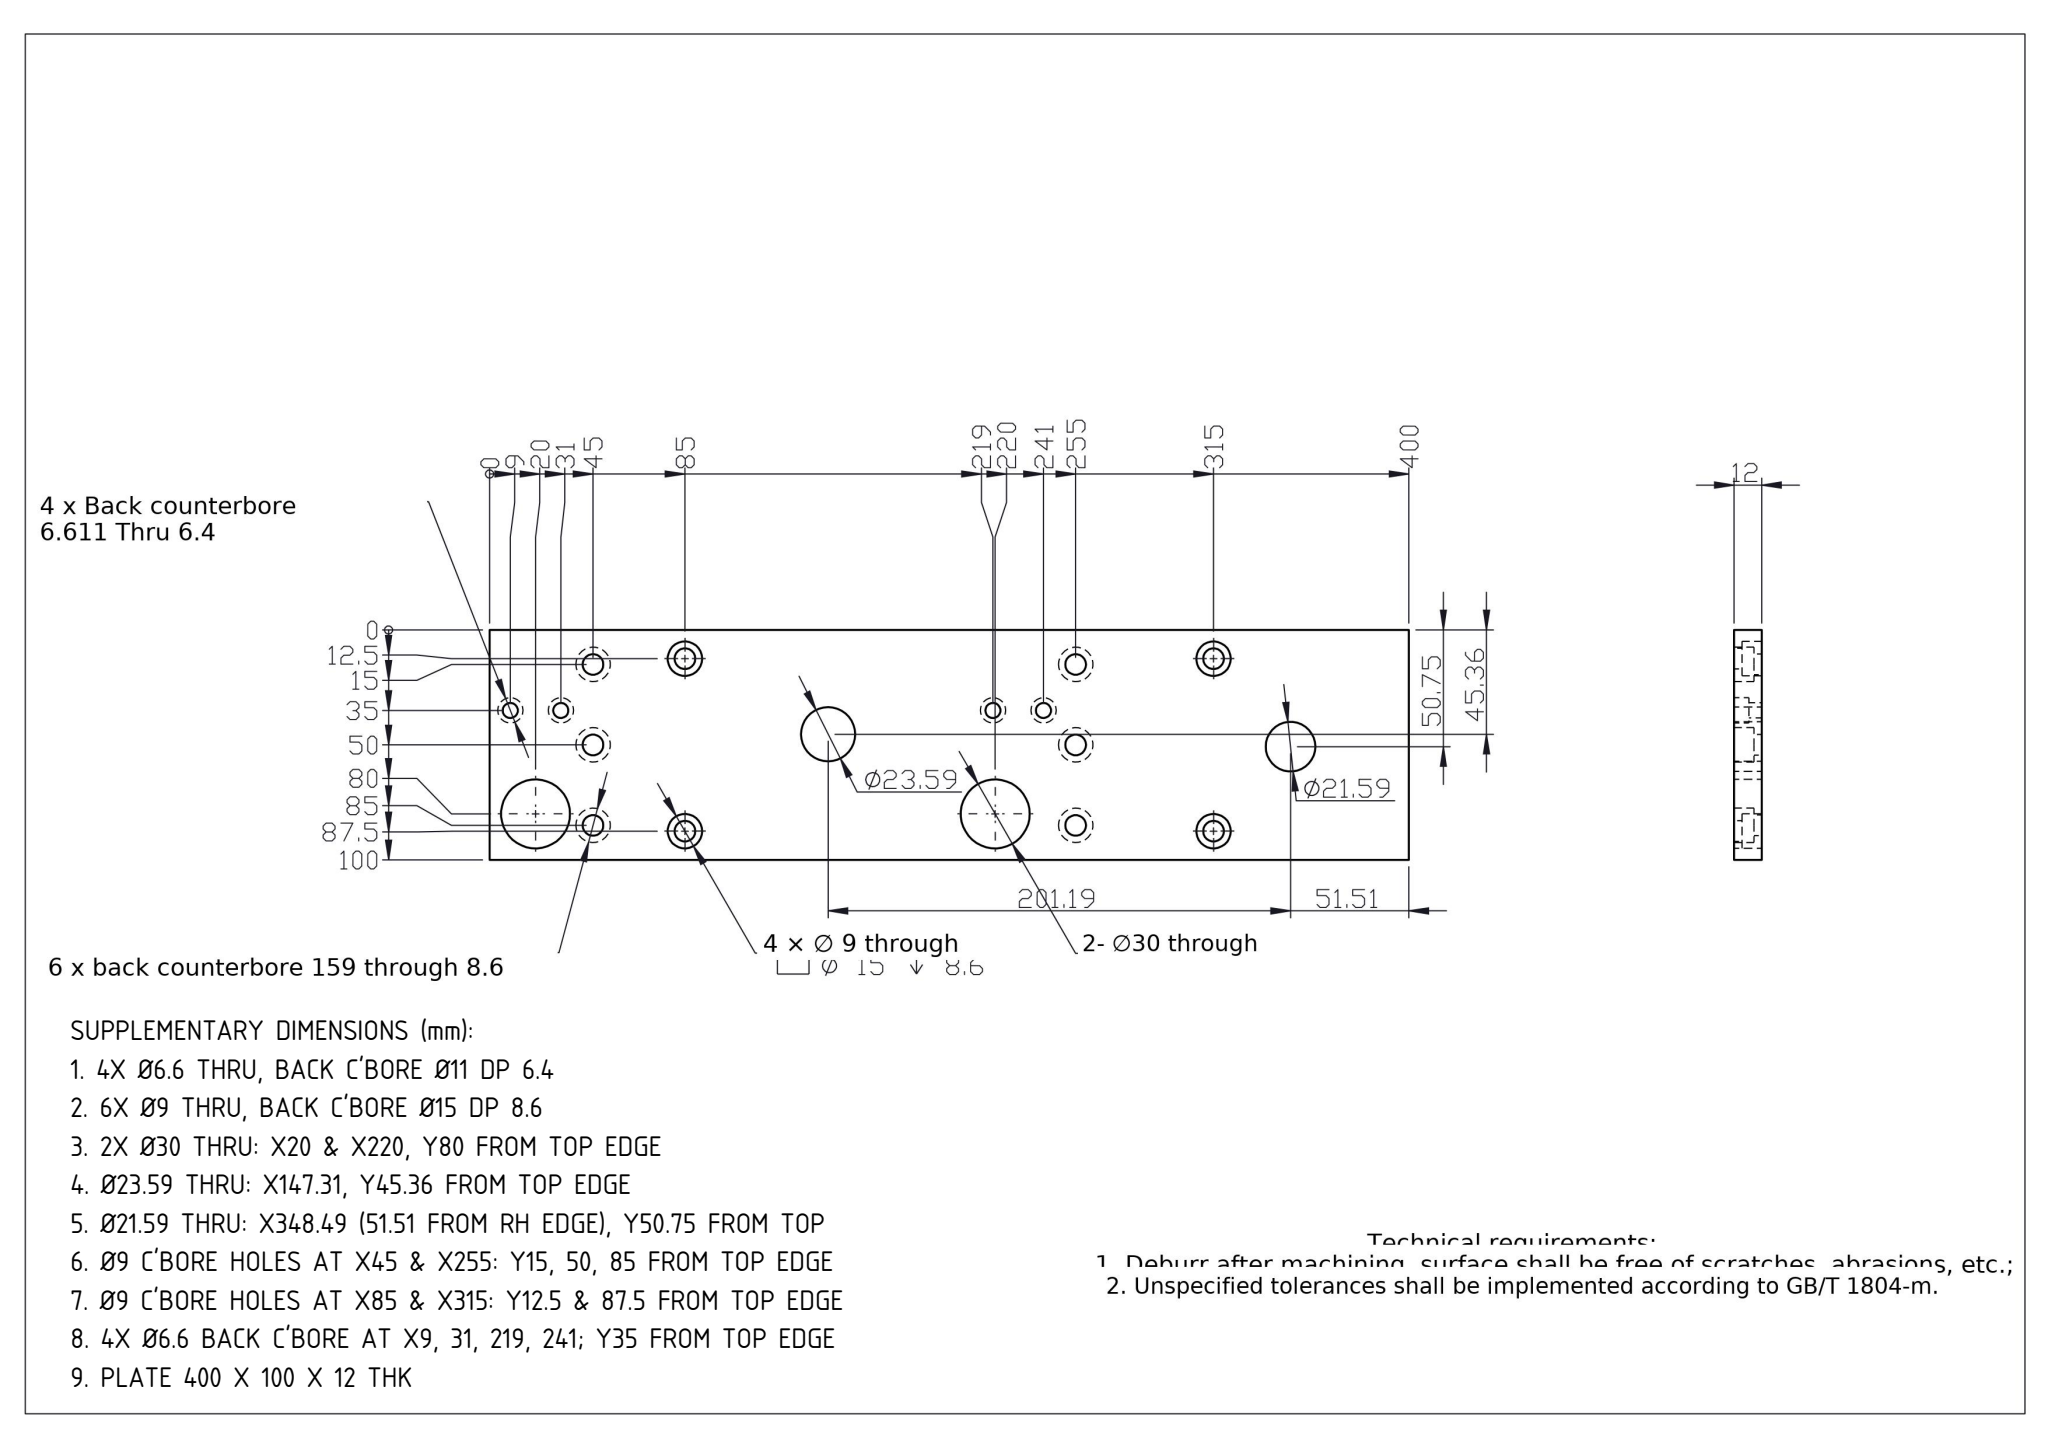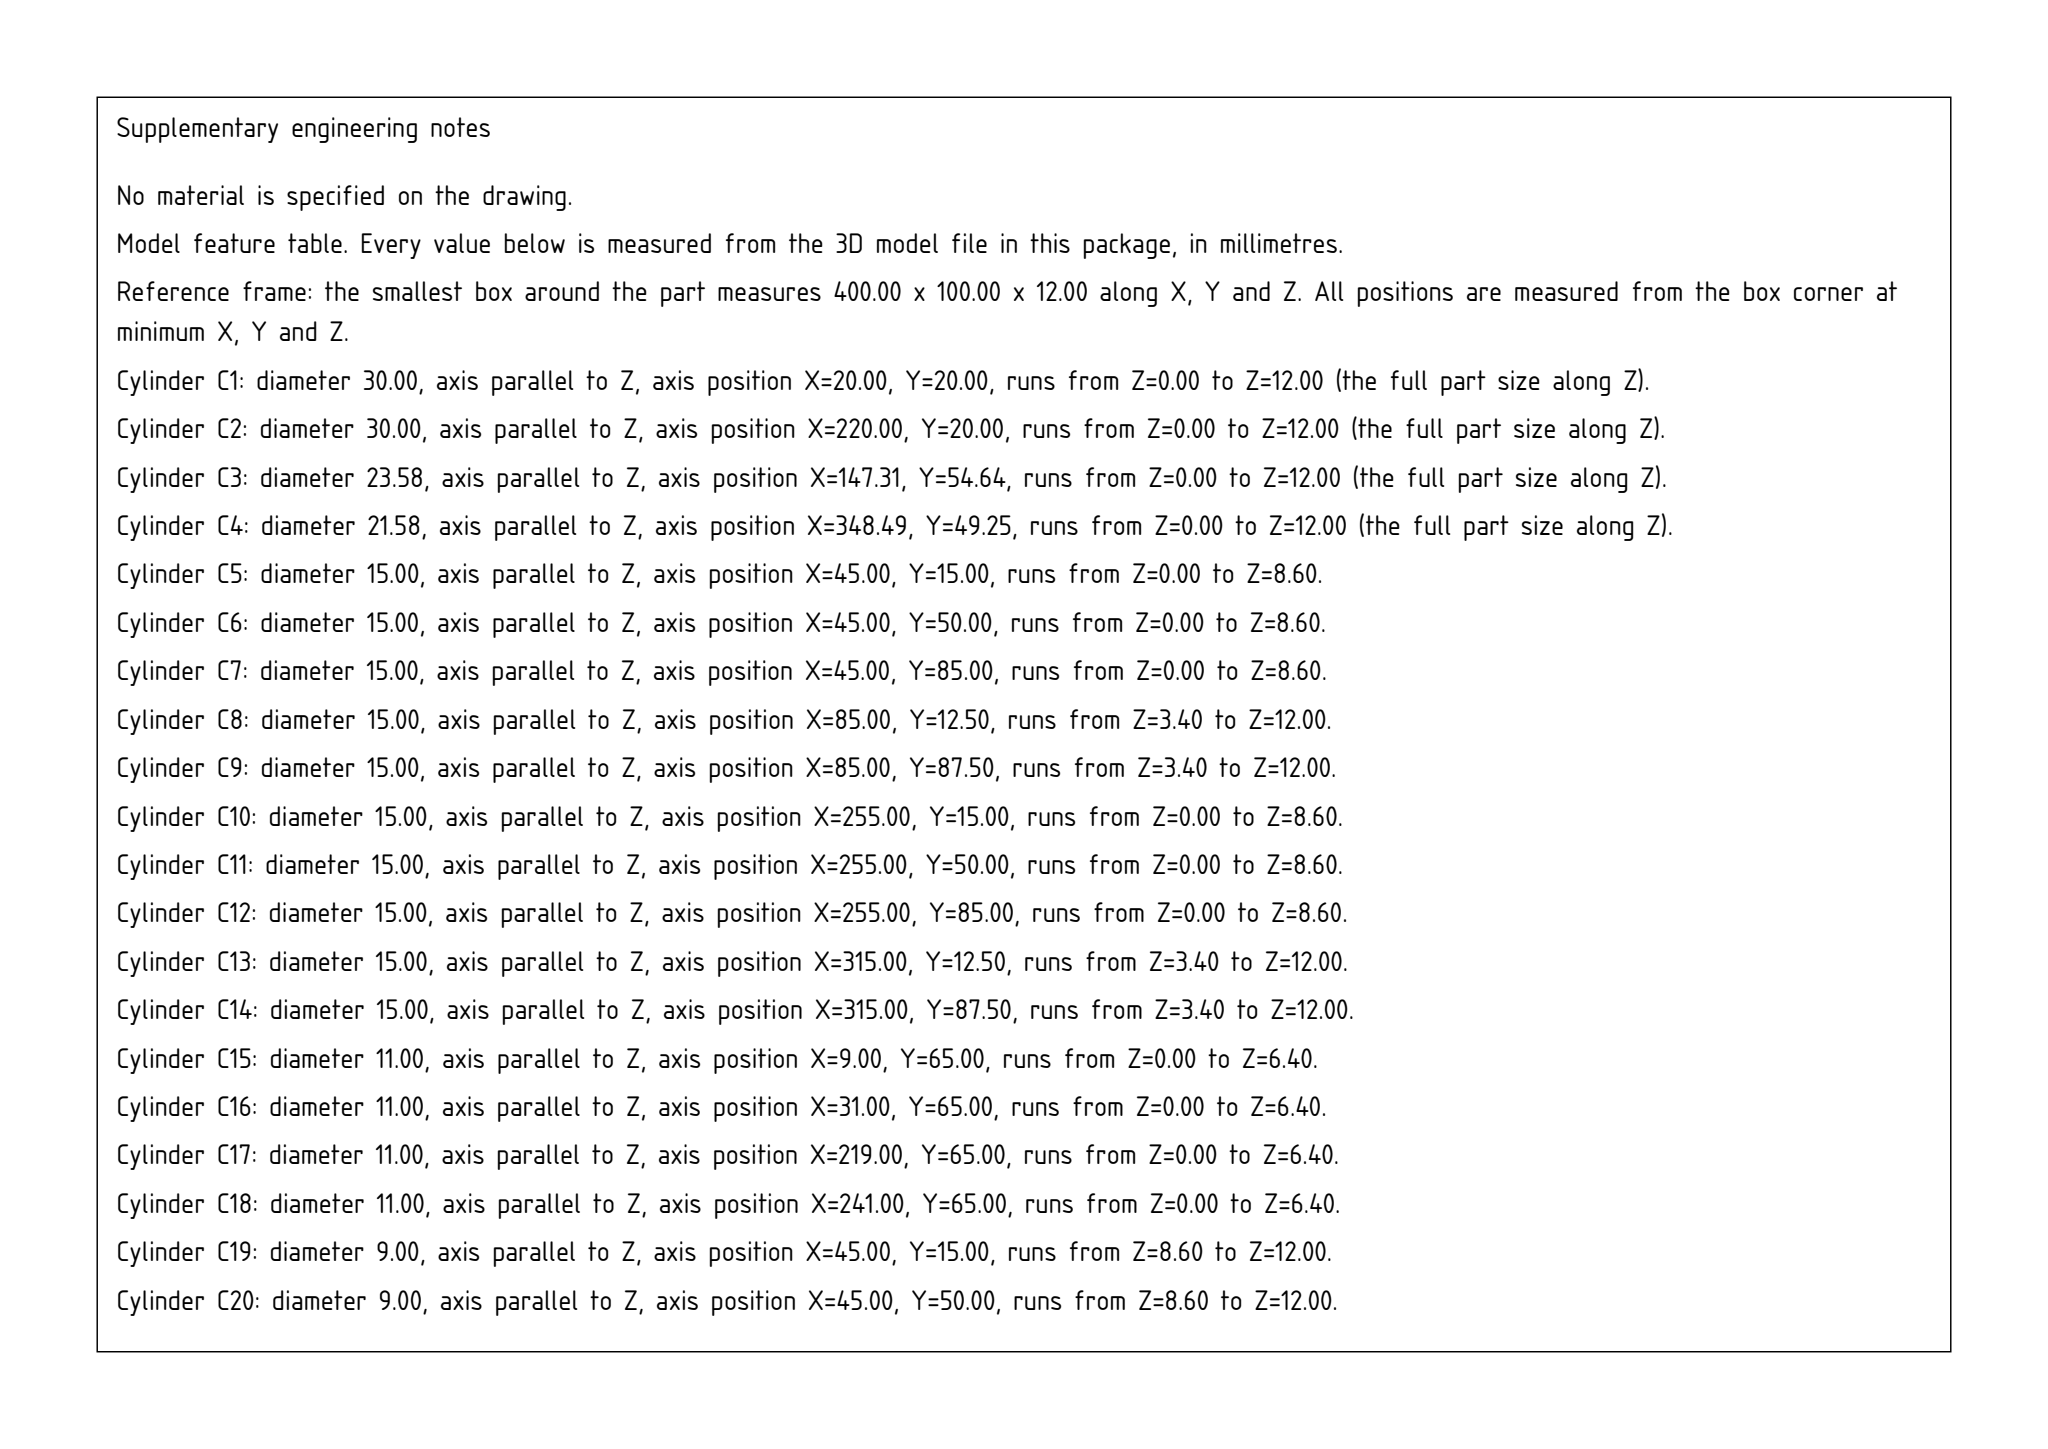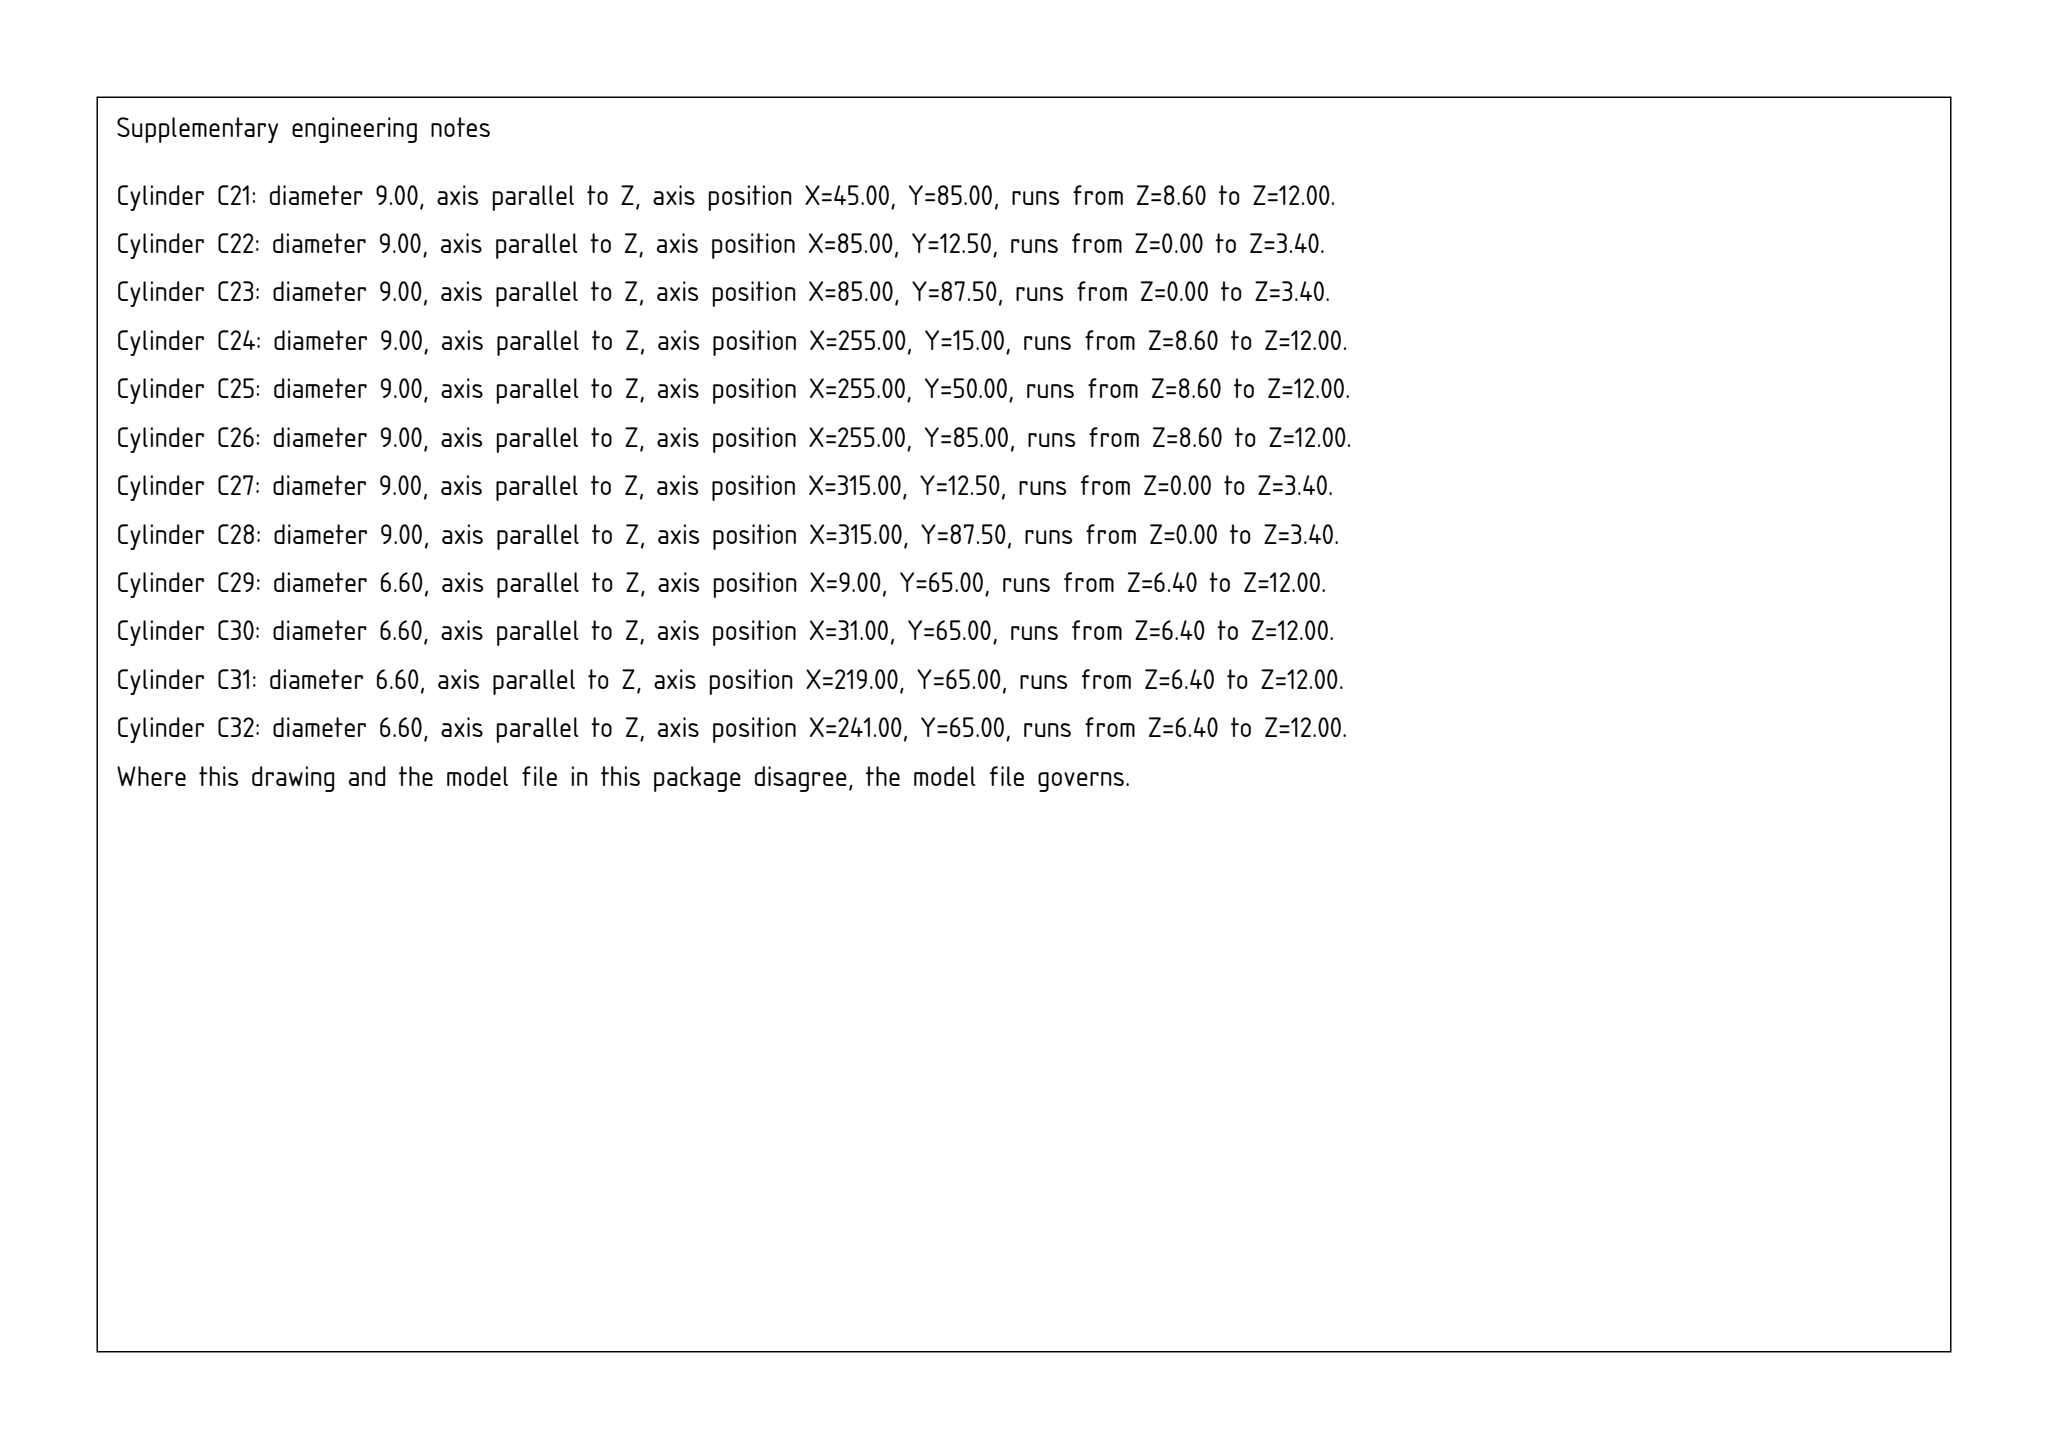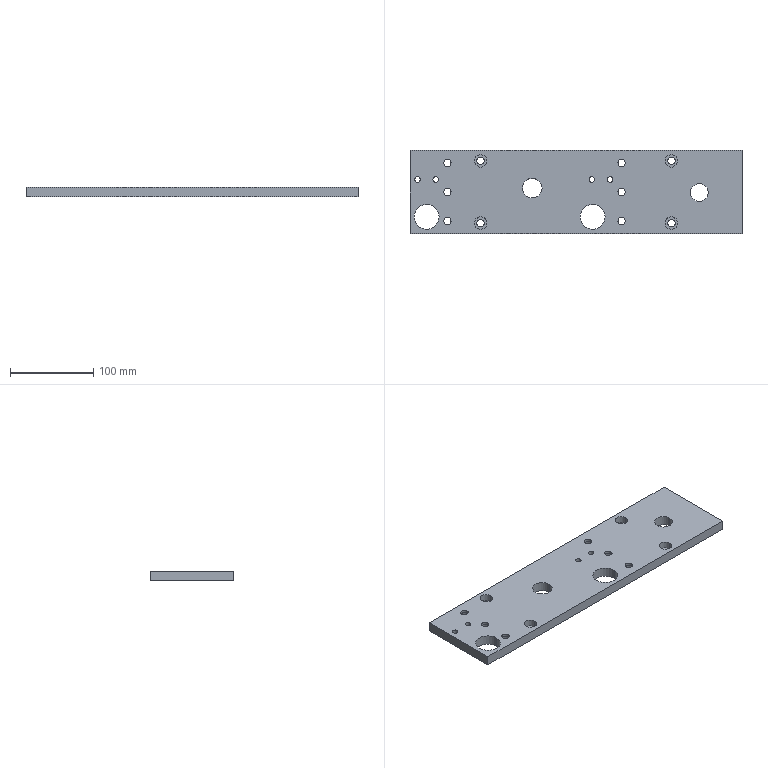Part | SolidWorks | mm | 1 solid | 84 faces | box 400 x 100 x 12 mm | volume 432839 mm3 | cylinder 64 | plane 20 | commonest cylinder face diameters 15 x20 9 x20 11 x8 6.6 x8 30 x4 23.589 x2 21.589 x2
build123d program:
from build123d import *

# Parameters (mm, degrees)
SKETCH1_W                                       = 400
SKETCH1_H                                       = 100
BOSS_EXTRUDE1_DEPTH                             = 12
M8_HEX_SOCKET_HEAD_CAP_SCREW_CBORE1_D           = 9
M8_HEX_SOCKET_HEAD_CAP_SCREW_CBORE1_CBORE_D     = 15
M8_HEX_SOCKET_HEAD_CAP_SCREW_CBORE1_CBORE_DEPTH = 8.6
M8_HEX_SOCKET_HEAD_CAP_SCREW_CBORE2_D           = 9
M8_HEX_SOCKET_HEAD_CAP_SCREW_CBORE2_CBORE_D     = 15
M8_HEX_SOCKET_HEAD_CAP_SCREW_CBORE2_CBORE_DEPTH = 8.6
M6_HEX_SOCKET_HEAD_CAP_SCREW_CBORE1_D           = 6.6
M6_HEX_SOCKET_HEAD_CAP_SCREW_CBORE1_CBORE_D     = 11
M6_HEX_SOCKET_HEAD_CAP_SCREW_CBORE1_CBORE_DEPTH = 6.4
SKETCH8_R                                       = 15
CUT_EXTRUDE1_DEPTH                              = 413.485
SKETCH9_R                                       = 11.794
SKETCH9_R_2                                     = 10.794
CUT_EXTRUDE2_DEPTH                              = 42


with BuildPart() as part:
    # Sketch1 → Boss-Extrude1 (new body)
    with BuildSketch(Plane.XY):
        with Locations((200, -50)):
            Rectangle(SKETCH1_W, SKETCH1_H)
    extrude(amount=BOSS_EXTRUDE1_DEPTH)

    # M8 Hex Socket Head Cap Screw CBORE1 (through all)
    with Locations(Plane.XY.offset(12)):
        with Locations((85, -12.5), (315, -12.5), (315, -87.5), (85, -87.5)):
            CounterBoreHole(M8_HEX_SOCKET_HEAD_CAP_SCREW_CBORE1_D / 2, M8_HEX_SOCKET_HEAD_CAP_SCREW_CBORE1_CBORE_D / 2, M8_HEX_SOCKET_HEAD_CAP_SCREW_CBORE1_CBORE_DEPTH)

    # M8 Hex Socket Head Cap Screw CBORE2 (through all)
    with Locations(Plane(origin=(0, 0, 0), x_dir=(-1, 0, 0), z_dir=(0, 0, -1))):
        with Locations((-45, -85), (-45, -50), (-45, -15), (-255, -15), (-255, -50), (-255, -85)):
            CounterBoreHole(M8_HEX_SOCKET_HEAD_CAP_SCREW_CBORE2_D / 2, M8_HEX_SOCKET_HEAD_CAP_SCREW_CBORE2_CBORE_D / 2, M8_HEX_SOCKET_HEAD_CAP_SCREW_CBORE2_CBORE_DEPTH)

    # M6 Hex Socket Head Cap Screw CBORE1 (through all)
    with Locations(Plane(origin=(0, 0, 0), x_dir=(-1, 0, 0), z_dir=(0, 0, -1))):
        with Locations((-9, -35), (-31, -35), (-219, -35), (-241, -35)):
            CounterBoreHole(M6_HEX_SOCKET_HEAD_CAP_SCREW_CBORE1_D / 2, M6_HEX_SOCKET_HEAD_CAP_SCREW_CBORE1_CBORE_D / 2, M6_HEX_SOCKET_HEAD_CAP_SCREW_CBORE1_CBORE_DEPTH)

    # Sketch8 → Cut-Extrude1 (cut, through all)
    with BuildSketch(Plane.XY.offset(12)):
        with Locations((20, -80)):
            Circle(SKETCH8_R)
        with Locations((220, -80)):
            Circle(SKETCH8_R)
    extrude(amount=-CUT_EXTRUDE1_DEPTH, mode=Mode.SUBTRACT)

    # Sketch9 → Cut-Extrude2 (cut)
    with BuildSketch(Plane.XY.offset(12)):
        with Locations((147.309, -45.36)):
            Circle(SKETCH9_R)
        with Locations((348.494, -50.748)):
            Circle(SKETCH9_R_2)
    extrude(amount=-CUT_EXTRUDE2_DEPTH, mode=Mode.SUBTRACT)


solid = part.part